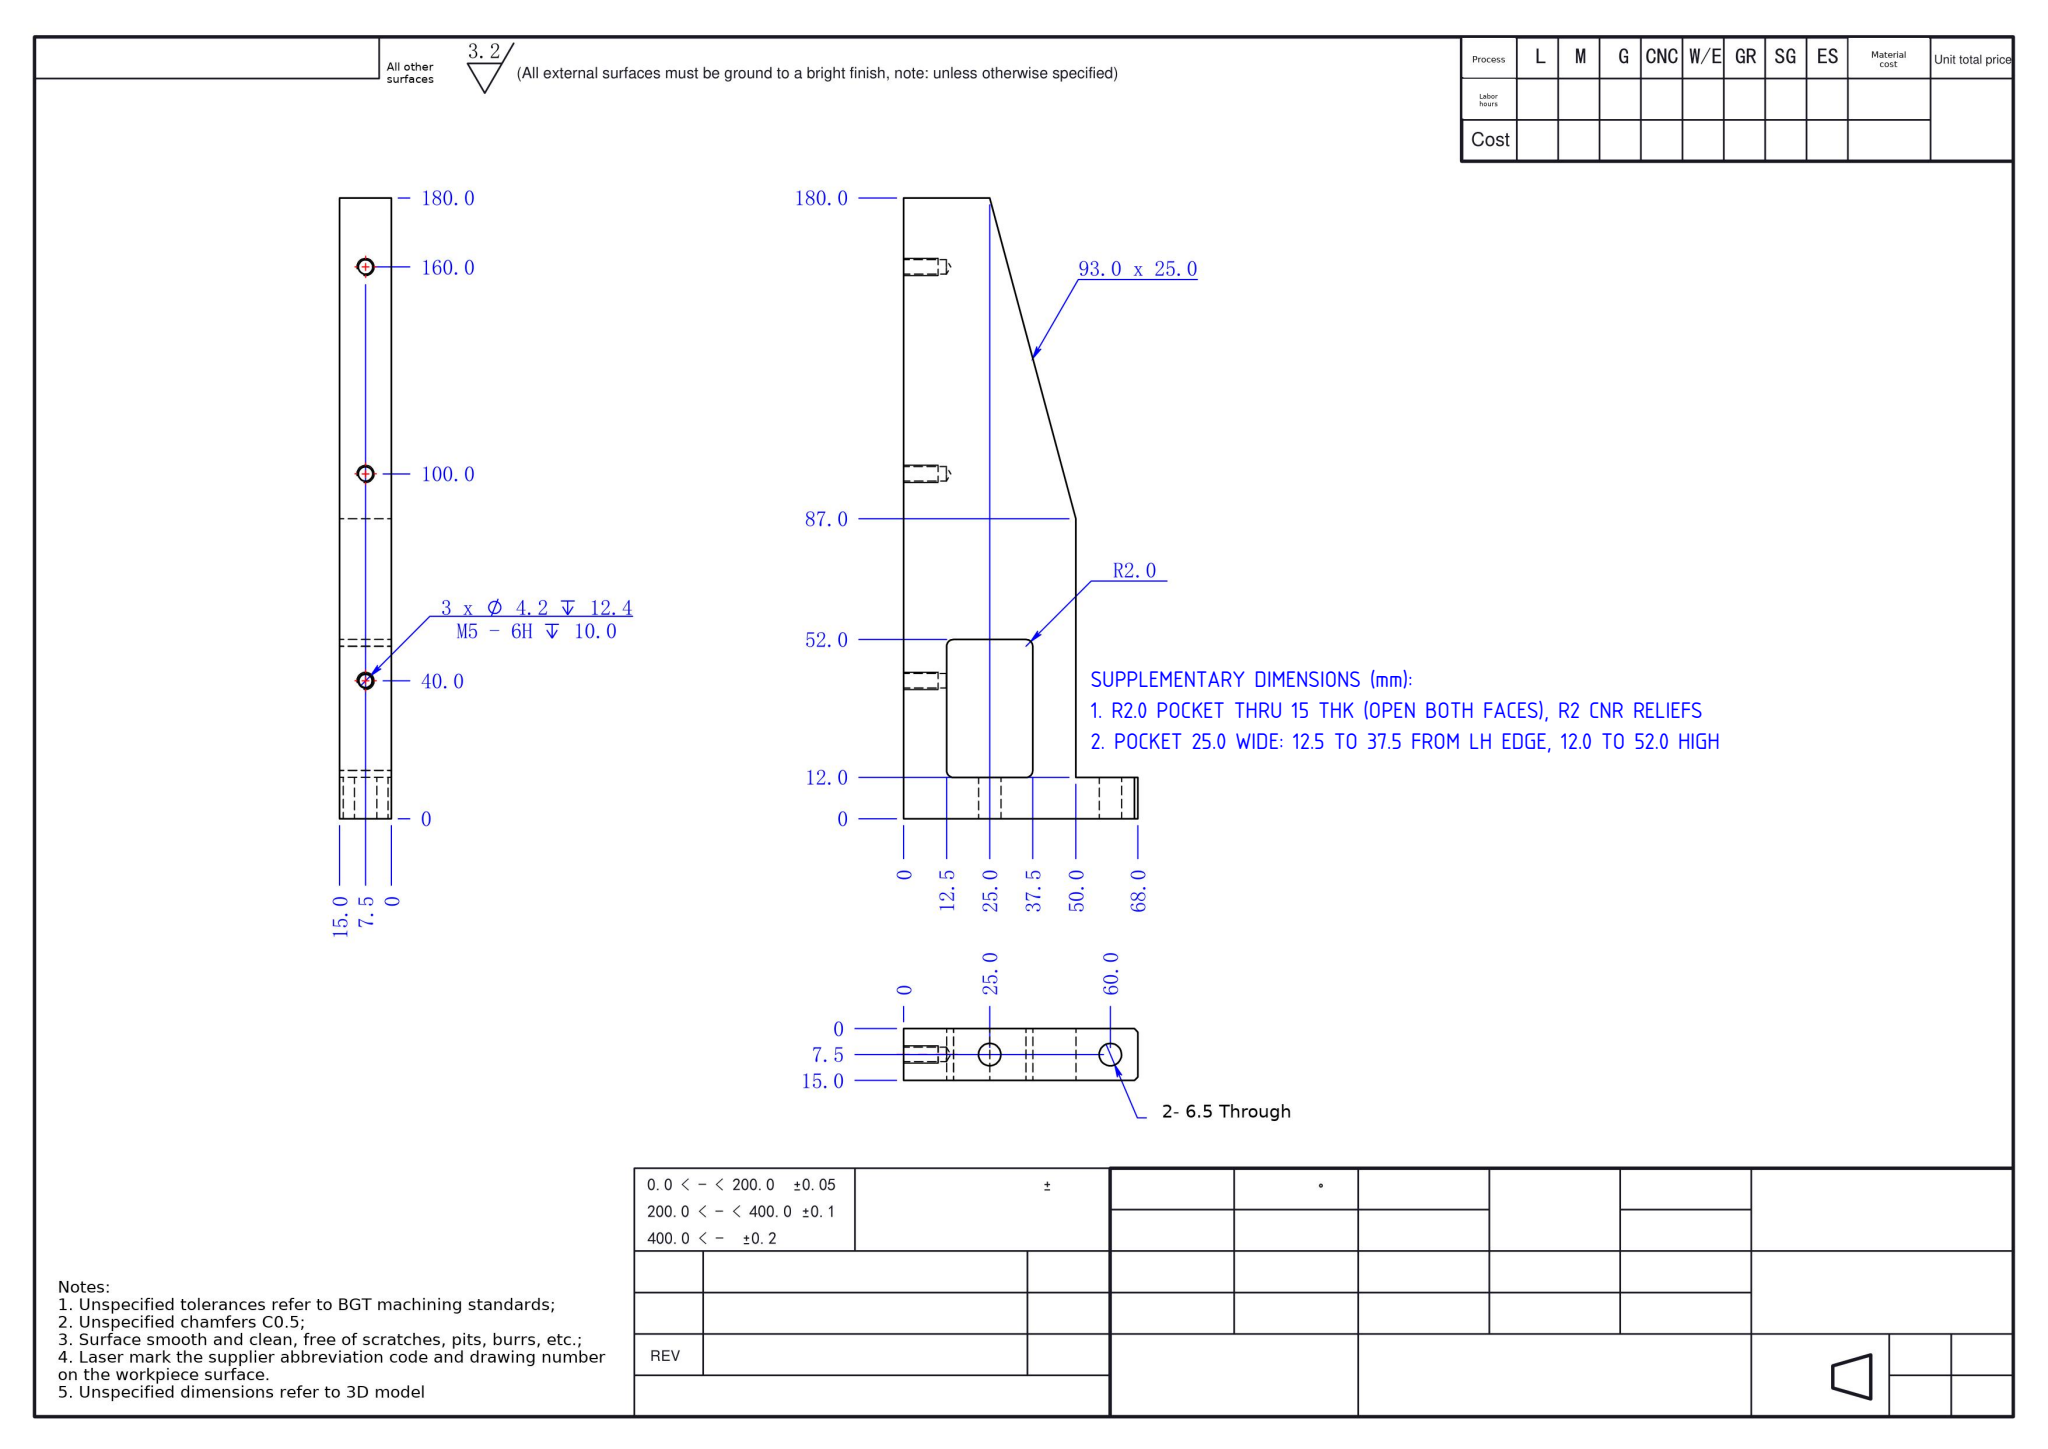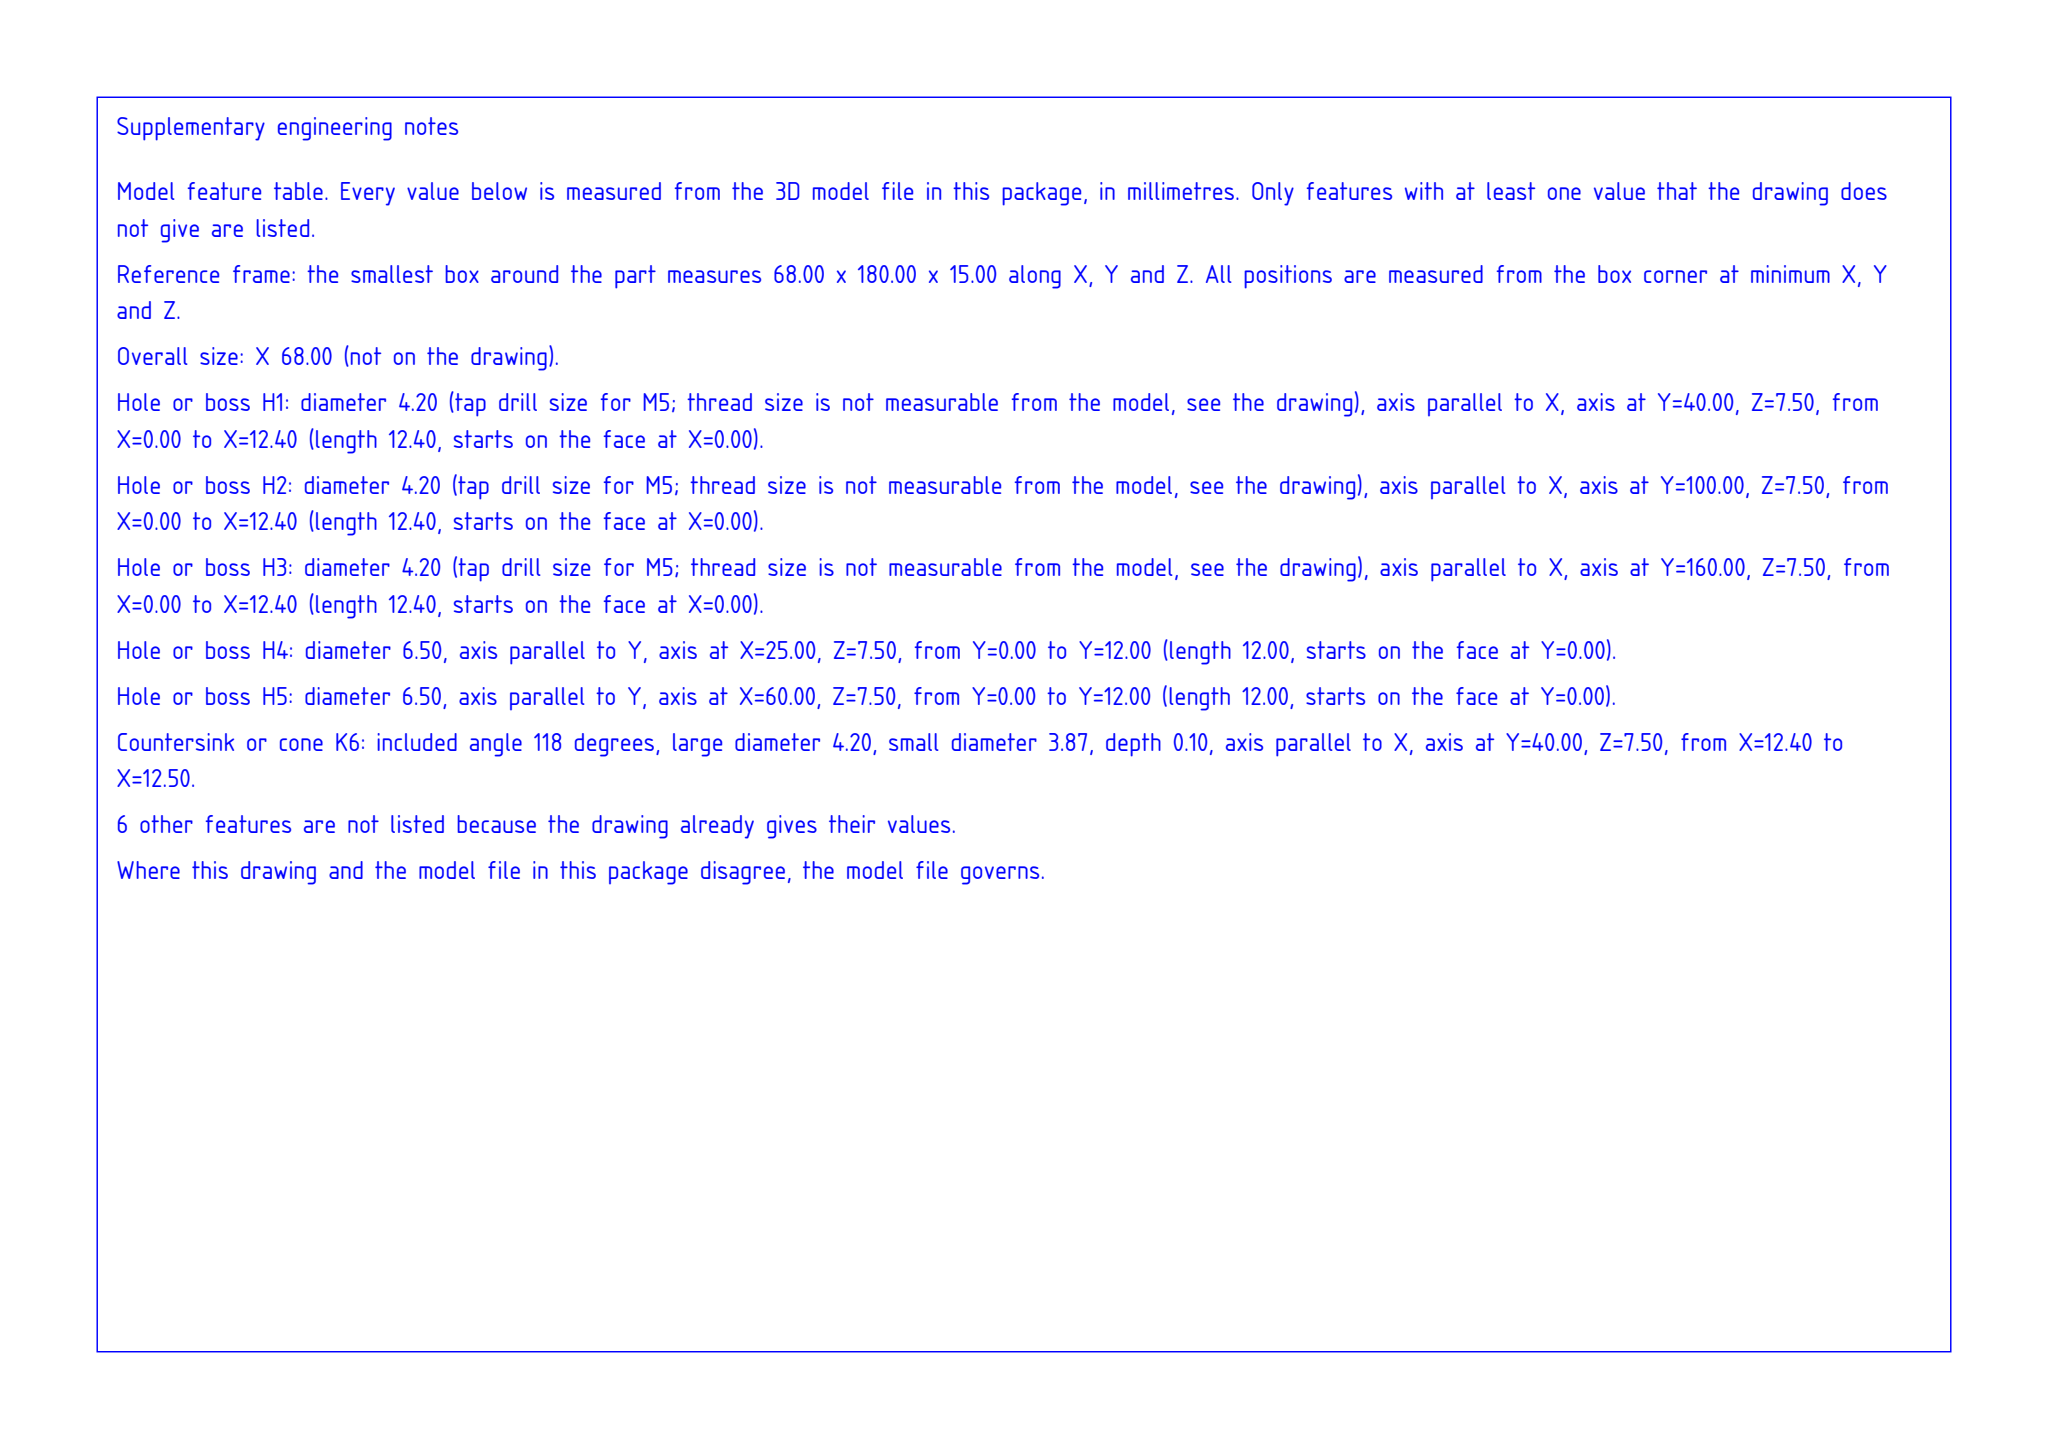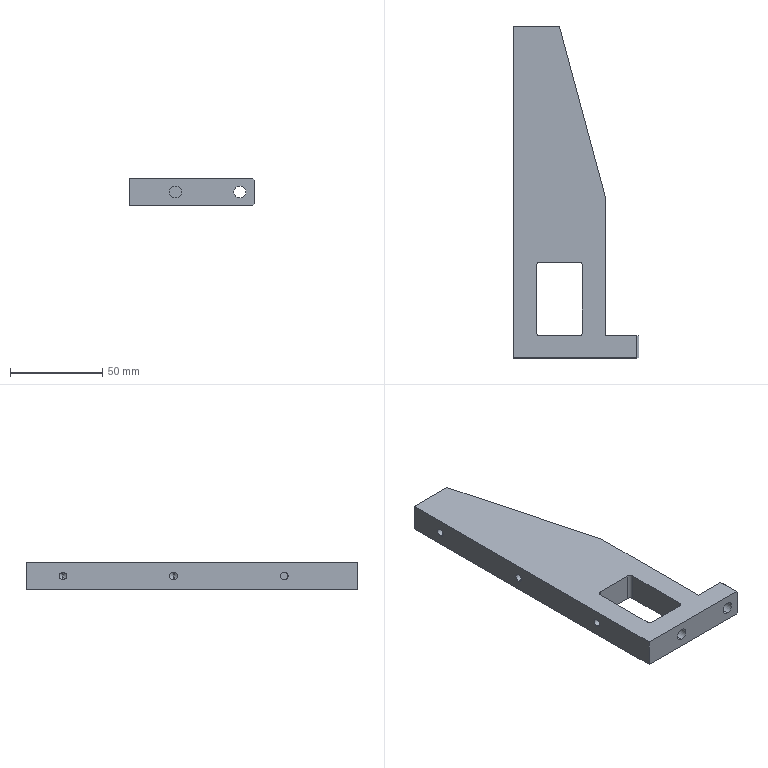Part | SolidWorks | mm | 1 solid | 35 faces | box 68 x 180 x 15 mm | volume 104513 mm3 | plane 15 | cylinder 14 | cone 6 | commonest cylinder face diameters 4.2 x6 6.5 x4 4 x4
build123d program:
from build123d import *

# Parameters (mm, degrees)
SKETCH1_W                      = 98
SKETCH1_H                      = 180
BOSS_EXTRUDE1_DEPTH            = 15
M5_TAPPED_HOLE1_D              = 4.2
M5_TAPPED_HOLE1_DEPTH          = 12.4
M5_TAPPED_HOLE1_TIP            = 1.262
CHAMFER1_SIZE                  = 10
M4_TAPPED_HOLE1_D              = 3.3
M4_TAPPED_HOLE1_DEPTH          = 10.1
M4_TAPPED_HOLE1_TIP            = 0.9914
CUT_EXTRUDE1_DEPTH             = 206.497
SKETCH11_W                     = 18
SKETCH11_H                     = 100
CUT_EXTRUDE2_DEPTH             = 194
F_6_5_6_5_DIAMETER_HOLE2_D     = 6.5
CHAMFER2_SIZE                  = 1
SKETCH14_W                     = 25
SKETCH14_H                     = 40
CUT_EXTRUDE3_DEPTH             = 194
FILLET1_R                      = 2
F_6_5_6_5_DIAMETER_HOLE1_D     = 6.5
F_6_5_6_5_DIAMETER_HOLE1_DEPTH = 30
F_6_5_6_5_DIAMETER_HOLE1_TIP   = 1.953


with BuildPart() as part:
    # Sketch1 → Boss-Extrude1 (new body)
    with BuildSketch(Plane.XY):
        with Locations((49, 90)):
            Rectangle(SKETCH1_W, SKETCH1_H)
    extrude(amount=BOSS_EXTRUDE1_DEPTH)

    # M5 Tapped Hole1
    with Locations(Plane.ZY):
        with Locations((7.5, 160), (7.5, 100), (7.5, 40)):
            Hole(M5_TAPPED_HOLE1_D / 2, depth=M5_TAPPED_HOLE1_DEPTH)
            with Locations((0, 0, -(M5_TAPPED_HOLE1_DEPTH + M5_TAPPED_HOLE1_TIP / 2))):  # 118° drill point
                Cone(0, M5_TAPPED_HOLE1_D / 2, M5_TAPPED_HOLE1_TIP, mode=Mode.SUBTRACT)

    # Chamfer1
    chamfer1_edges = [part.edges().sort_by_distance(p)[0] for p in [
        (98, 180, 7.5),
    ]]
    chamfer(chamfer1_edges, length=CHAMFER1_SIZE)

    # M4 Tapped Hole1
    with Locations(Plane(origin=(0, 180, 0), x_dir=(1, 0, 0), z_dir=(0, 1, 0))):
        with Locations((105, -7.5), (70, -7.5), (35, -7.5)):
            Hole(M4_TAPPED_HOLE1_D / 2, depth=M4_TAPPED_HOLE1_DEPTH)
            with Locations((0, 0, -(M4_TAPPED_HOLE1_DEPTH + M4_TAPPED_HOLE1_TIP / 2))):  # 118° drill point
                Cone(0, M4_TAPPED_HOLE1_D / 2, M4_TAPPED_HOLE1_TIP, mode=Mode.SUBTRACT)

    # Sketch8 → Cut-Extrude1 (cut, through all)
    with BuildSketch(Plane.XY.offset(15)):
        Polygon((68, 0), (68, 20), (25, 180), (88, 180), (98, 170), (98, 0), align=None)
    extrude(amount=-CUT_EXTRUDE1_DEPTH, mode=Mode.SUBTRACT)

    # Sketch11 → Cut-Extrude2 (cut, through all)
    with BuildSketch(Plane.XY.offset(15)):
        with Locations((59, 62)):
            Rectangle(SKETCH11_W, SKETCH11_H)
    extrude(amount=-CUT_EXTRUDE2_DEPTH, mode=Mode.SUBTRACT)

    # 6.5 _6.5_ Diameter Hole2 (through all)
    with Locations(Plane(origin=(0, 12, 0), x_dir=(1, 0, 0), z_dir=(0, 1, 0))):
        with Locations((60, -7.5)):
            Hole(F_6_5_6_5_DIAMETER_HOLE2_D / 2)

    # Chamfer2
    chamfer2_edges = [part.edges().sort_by_distance(p)[0] for p in [
        (68, 6, 15),
        (68, 6, 0),
    ]]
    chamfer(chamfer2_edges, length=CHAMFER2_SIZE)

    # Sketch14 → Cut-Extrude3 (cut, through all)
    with BuildSketch(Plane.XY.offset(15)):
        with Locations((25, 32)):
            Rectangle(SKETCH14_W, SKETCH14_H)
    extrude(amount=-CUT_EXTRUDE3_DEPTH, mode=Mode.SUBTRACT)

    # Fillet1
    fillet1_edges = [part.edges().sort_by_distance(p)[0] for p in [
        (12.5, 12, 7.5),
        (12.5, 52, 7.5),
        (37.5, 52, 7.5),
        (37.5, 12, 7.5),
    ]]
    fillet(fillet1_edges, radius=FILLET1_R)

    # 6.5 _6.5_ Diameter Hole1
    with Locations(Plane(origin=(0, 0, 0), x_dir=(-1, 0, 0), z_dir=(0, -1, 0))):
        with Locations((-25, -7.5)):
            Hole(F_6_5_6_5_DIAMETER_HOLE1_D / 2, depth=F_6_5_6_5_DIAMETER_HOLE1_DEPTH)
            with Locations((0, 0, -(F_6_5_6_5_DIAMETER_HOLE1_DEPTH + F_6_5_6_5_DIAMETER_HOLE1_TIP / 2))):  # 118° drill point
                Cone(0, F_6_5_6_5_DIAMETER_HOLE1_D / 2, F_6_5_6_5_DIAMETER_HOLE1_TIP, mode=Mode.SUBTRACT)


solid = part.part